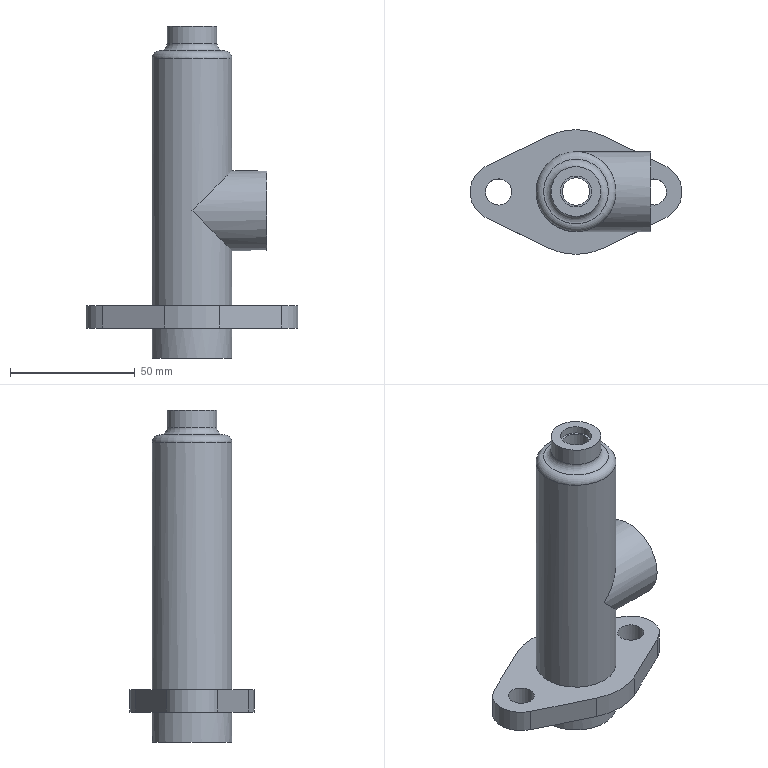Component | NX | CYLINDER_BODY | 1 solid | 37 faces | volume 85652 mm3 | cylinder 17 | plane 13 | cone 5 | torus 2 | commonest cylinder face diameters 32 x3 3.5 x2 50 x2 23 x2 10.5 x2 21 x1 12.5 x1 11 x1